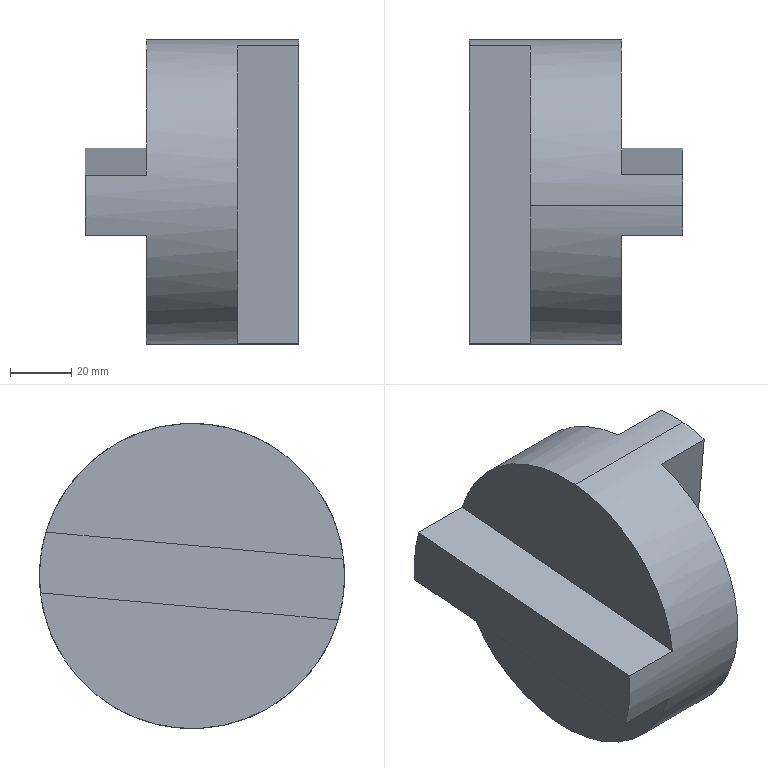Component | SolidWorks | CouplerAssembly-1_MiddleCoupler-1 | 1 solid | 12 faces | volume 315083 mm3 | plane 10 | cylinder 2 | commonest cylinder face diameters 100 x2